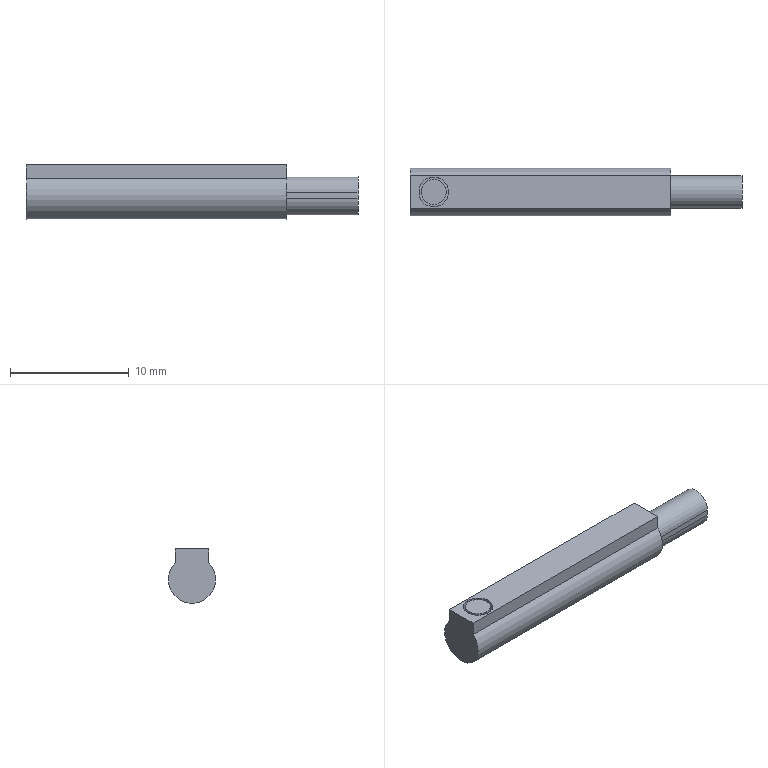Component | SolidWorks | MGPM20-20Z-M9P-1_D_M9P_MGP_Z_6-2 | 1 solid | 17 faces | box 28 x 4 x 4.6 mm | volume 365 mm3 | plane 10 | cylinder 7 | commonest cylinder face diameters 2.7 x2 2.5 x2 2.1 x2 4 x1
STEP:
#1=COLOUR_RGB('',0.7922,0.8196,0.9333);
#2=FILL_AREA_STYLE_COLOUR('',#1);
#3=FILL_AREA_STYLE('',(#2));
#4=SURFACE_STYLE_FILL_AREA(#3);
#5=SURFACE_SIDE_STYLE('',(#4));
#6=SURFACE_STYLE_USAGE(.BOTH.,#5);
#7=PRESENTATION_STYLE_ASSIGNMENT((#6));
#8=CARTESIAN_POINT('',(2.517,1.889,2.967));
#9=VERTEX_POINT('',#8);
#10=CARTESIAN_POINT('',(2.517,1.988,2.967));
#11=VERTEX_POINT('',#10);
#12=CARTESIAN_POINT('',(2.517,1.938,2.967));
#13=DIRECTION('',(0.,0.,1.));
#14=DIRECTION('',(0.,-1.,0.));
#15=AXIS2_PLACEMENT_3D('',#12,#13,#14);
#16=CIRCLE('',#15,0.04921);
#17=EDGE_CURVE('',#9,#11,#16,.T.);
#18=ORIENTED_EDGE('',*,*,#17,.F.);
#19=CARTESIAN_POINT('',(2.517,1.938,2.967));
#20=DIRECTION('',(0.,0.,1.));
#21=DIRECTION('',(0.,-1.,0.));
#22=AXIS2_PLACEMENT_3D('',#19,#20,#21);
#23=CIRCLE('',#22,0.04921);
#24=EDGE_CURVE('',#11,#9,#23,.T.);
#25=ORIENTED_EDGE('',*,*,#24,.F.);
#26=EDGE_LOOP('',(#18,#25));
#27=FACE_BOUND('',#26,.T.);
#28=CARTESIAN_POINT('',(2.438,1.883,2.967));
#29=VERTEX_POINT('',#28);
#30=CARTESIAN_POINT('',(2.438,1.994,2.967));
#31=VERTEX_POINT('',#30);
#32=CARTESIAN_POINT('',(2.438,1.883,2.967));
#33=DIRECTION('',(-0.,1.,-0.));
#34=VECTOR('',#33,39.37);
#35=LINE('',#32,#34);
#36=EDGE_CURVE('',#29,#31,#35,.T.);
#37=ORIENTED_EDGE('',*,*,#36,.F.);
#38=CARTESIAN_POINT('',(3.304,1.883,2.967));
#39=VERTEX_POINT('',#38);
#40=CARTESIAN_POINT('',(3.304,1.883,2.967));
#41=DIRECTION('',(-1.,-0.,0.));
#42=VECTOR('',#41,39.37);
#43=LINE('',#40,#42);
#44=EDGE_CURVE('',#39,#29,#43,.T.);
#45=ORIENTED_EDGE('',*,*,#44,.F.);
#46=CARTESIAN_POINT('',(3.304,1.994,2.967));
#47=VERTEX_POINT('',#46);
#48=CARTESIAN_POINT('',(3.304,1.883,2.967));
#49=DIRECTION('',(-0.,1.,-0.));
#50=VECTOR('',#49,39.37);
#51=LINE('',#48,#50);
#52=EDGE_CURVE('',#39,#47,#51,.T.);
#53=ORIENTED_EDGE('',*,*,#52,.T.);
#54=CARTESIAN_POINT('',(3.304,1.994,2.967));
#55=DIRECTION('',(-1.,-0.,0.));
#56=VECTOR('',#55,39.37);
#57=LINE('',#54,#56);
#58=EDGE_CURVE('',#47,#31,#57,.T.);
#59=ORIENTED_EDGE('',*,*,#58,.T.);
#60=EDGE_LOOP('',(#37,#45,#53,#59));
#61=FACE_OUTER_BOUND('',#60,.T.);
#62=CARTESIAN_POINT('',(3.304,1.883,2.967));
#63=DIRECTION('',(0.,0.,1.));
#64=DIRECTION('',(-1.,-0.,0.));
#65=AXIS2_PLACEMENT_3D('',#62,#63,#64);
#66=PLANE('',#65);
#67=ADVANCED_FACE('',(#27,#61),#66,.T.);
#68=CARTESIAN_POINT('',(2.438,1.994,2.921));
#69=VERTEX_POINT('',#68);
#70=CARTESIAN_POINT('',(2.438,1.994,2.967));
#71=DIRECTION('',(-0.,-0.,-1.));
#72=VECTOR('',#71,39.37);
#73=LINE('',#70,#72);
#74=EDGE_CURVE('',#31,#69,#73,.T.);
#75=ORIENTED_EDGE('',*,*,#74,.F.);
#76=ORIENTED_EDGE('',*,*,#58,.F.);
#77=CARTESIAN_POINT('',(3.304,1.994,2.921));
#78=VERTEX_POINT('',#77);
#79=CARTESIAN_POINT('',(3.304,1.994,2.967));
#80=DIRECTION('',(-0.,-0.,-1.));
#81=VECTOR('',#80,39.37);
#82=LINE('',#79,#81);
#83=EDGE_CURVE('',#47,#78,#82,.T.);
#84=ORIENTED_EDGE('',*,*,#83,.T.);
#85=CARTESIAN_POINT('',(3.304,1.994,2.921));
#86=DIRECTION('',(-1.,-0.,0.));
#87=VECTOR('',#86,39.37);
#88=LINE('',#85,#87);
#89=EDGE_CURVE('',#78,#69,#88,.T.);
#90=ORIENTED_EDGE('',*,*,#89,.T.);
#91=EDGE_LOOP('',(#75,#76,#84,#90));
#92=FACE_OUTER_BOUND('',#91,.T.);
#93=CARTESIAN_POINT('',(3.304,1.994,2.967));
#94=DIRECTION('',(-0.,1.,-0.));
#95=DIRECTION('',(-1.,-0.,0.));
#96=AXIS2_PLACEMENT_3D('',#93,#94,#95);
#97=PLANE('',#96);
#98=ADVANCED_FACE('',(#92),#97,.T.);
#99=CARTESIAN_POINT('',(2.438,1.883,2.921));
#100=VERTEX_POINT('',#99);
#101=CARTESIAN_POINT('',(2.438,1.938,2.865));
#102=DIRECTION('',(-1.,-0.,0.));
#103=DIRECTION('',(0.,-1.,0.));
#104=AXIS2_PLACEMENT_3D('',#101,#102,#103);
#105=CIRCLE('',#104,0.07874);
#106=EDGE_CURVE('',#69,#100,#105,.T.);
#107=ORIENTED_EDGE('',*,*,#106,.F.);
#108=ORIENTED_EDGE('',*,*,#89,.F.);
#109=CARTESIAN_POINT('',(3.304,1.883,2.921));
#110=VERTEX_POINT('',#109);
#111=CARTESIAN_POINT('',(3.304,1.938,2.865));
#112=DIRECTION('',(-1.,-0.,0.));
#113=DIRECTION('',(0.,-1.,0.));
#114=AXIS2_PLACEMENT_3D('',#111,#112,#113);
#115=CIRCLE('',#114,0.07874);
#116=EDGE_CURVE('',#78,#110,#115,.T.);
#117=ORIENTED_EDGE('',*,*,#116,.T.);
#118=CARTESIAN_POINT('',(3.304,1.883,2.921));
#119=DIRECTION('',(-1.,-0.,0.));
#120=VECTOR('',#119,39.37);
#121=LINE('',#118,#120);
#122=EDGE_CURVE('',#110,#100,#121,.T.);
#123=ORIENTED_EDGE('',*,*,#122,.T.);
#124=EDGE_LOOP('',(#107,#108,#117,#123));
#125=FACE_OUTER_BOUND('',#124,.T.);
#126=CARTESIAN_POINT('',(3.304,1.938,2.865));
#127=DIRECTION('',(1.,0.,-0.));
#128=DIRECTION('',(0.,0.,1.));
#129=AXIS2_PLACEMENT_3D('',#126,#127,#128);
#130=CYLINDRICAL_SURFACE('',#129,0.07874);
#131=ADVANCED_FACE('',(#125),#130,.T.);
#132=CARTESIAN_POINT('',(2.438,1.883,2.921));
#133=DIRECTION('',(0.,0.,1.));
#134=VECTOR('',#133,39.37);
#135=LINE('',#132,#134);
#136=EDGE_CURVE('',#100,#29,#135,.T.);
#137=ORIENTED_EDGE('',*,*,#136,.F.);
#138=ORIENTED_EDGE('',*,*,#122,.F.);
#139=CARTESIAN_POINT('',(3.304,1.883,2.921));
#140=DIRECTION('',(0.,0.,1.));
#141=VECTOR('',#140,39.37);
#142=LINE('',#139,#141);
#143=EDGE_CURVE('',#110,#39,#142,.T.);
#144=ORIENTED_EDGE('',*,*,#143,.T.);
#145=ORIENTED_EDGE('',*,*,#44,.T.);
#146=EDGE_LOOP('',(#137,#138,#144,#145));
#147=FACE_OUTER_BOUND('',#146,.T.);
#148=CARTESIAN_POINT('',(3.304,1.883,2.921));
#149=DIRECTION('',(0.,-1.,0.));
#150=DIRECTION('',(1.,0.,-0.));
#151=AXIS2_PLACEMENT_3D('',#148,#149,#150);
#152=PLANE('',#151);
#153=ADVANCED_FACE('',(#147),#152,.T.);
#154=CARTESIAN_POINT('',(3.304,1.885,2.875));
#155=VERTEX_POINT('',#154);
#156=CARTESIAN_POINT('',(3.304,1.992,2.875));
#157=VERTEX_POINT('',#156);
#158=CARTESIAN_POINT('',(3.304,1.938,2.875));
#159=DIRECTION('',(-1.,-0.,0.));
#160=DIRECTION('',(0.,-1.,0.));
#161=AXIS2_PLACEMENT_3D('',#158,#159,#160);
#162=CIRCLE('',#161,0.05315);
#163=EDGE_CURVE('',#155,#157,#162,.T.);
#164=ORIENTED_EDGE('',*,*,#163,.T.);
#165=CARTESIAN_POINT('',(3.304,1.992,2.855));
#166=VERTEX_POINT('',#165);
#167=CARTESIAN_POINT('',(3.304,1.992,2.875));
#168=DIRECTION('',(-0.,-0.,-1.));
#169=VECTOR('',#168,39.37);
#170=LINE('',#167,#169);
#171=EDGE_CURVE('',#157,#166,#170,.T.);
#172=ORIENTED_EDGE('',*,*,#171,.T.);
#173=CARTESIAN_POINT('',(3.304,1.885,2.855));
#174=VERTEX_POINT('',#173);
#175=CARTESIAN_POINT('',(3.304,1.938,2.855));
#176=DIRECTION('',(-1.,-0.,0.));
#177=DIRECTION('',(0.,-1.,0.));
#178=AXIS2_PLACEMENT_3D('',#175,#176,#177);
#179=CIRCLE('',#178,0.05315);
#180=EDGE_CURVE('',#166,#174,#179,.T.);
#181=ORIENTED_EDGE('',*,*,#180,.T.);
#182=CARTESIAN_POINT('',(3.304,1.885,2.855));
#183=DIRECTION('',(0.,0.,1.));
#184=VECTOR('',#183,39.37);
#185=LINE('',#182,#184);
#186=EDGE_CURVE('',#174,#155,#185,.T.);
#187=ORIENTED_EDGE('',*,*,#186,.T.);
#188=EDGE_LOOP('',(#164,#172,#181,#187));
#189=FACE_BOUND('',#188,.T.);
#190=ORIENTED_EDGE('',*,*,#83,.F.);
#191=ORIENTED_EDGE('',*,*,#52,.F.);
#192=ORIENTED_EDGE('',*,*,#143,.F.);
#193=ORIENTED_EDGE('',*,*,#116,.F.);
#194=EDGE_LOOP('',(#190,#191,#192,#193));
#195=FACE_OUTER_BOUND('',#194,.T.);
#196=CARTESIAN_POINT('',(3.304,1.938,2.865));
#197=DIRECTION('',(-1.,-0.,0.));
#198=DIRECTION('',(0.,-1.,0.));
#199=AXIS2_PLACEMENT_3D('',#196,#197,#198);
#200=PLANE('',#199);
#201=ADVANCED_FACE('',(#189,#195),#200,.F.);
#202=ORIENTED_EDGE('',*,*,#186,.F.);
#203=CARTESIAN_POINT('',(3.54,1.885,2.855));
#204=VERTEX_POINT('',#203);
#205=CARTESIAN_POINT('',(3.54,1.885,2.855));
#206=DIRECTION('',(-1.,-0.,0.));
#207=VECTOR('',#206,39.37);
#208=LINE('',#205,#207);
#209=EDGE_CURVE('',#204,#174,#208,.T.);
#210=ORIENTED_EDGE('',*,*,#209,.F.);
#211=CARTESIAN_POINT('',(3.54,1.885,2.875));
#212=VERTEX_POINT('',#211);
#213=CARTESIAN_POINT('',(3.54,1.885,2.855));
#214=DIRECTION('',(0.,0.,1.));
#215=VECTOR('',#214,39.37);
#216=LINE('',#213,#215);
#217=EDGE_CURVE('',#204,#212,#216,.T.);
#218=ORIENTED_EDGE('',*,*,#217,.T.);
#219=CARTESIAN_POINT('',(3.54,1.885,2.875));
#220=DIRECTION('',(-1.,-0.,0.));
#221=VECTOR('',#220,39.37);
#222=LINE('',#219,#221);
#223=EDGE_CURVE('',#212,#155,#222,.T.);
#224=ORIENTED_EDGE('',*,*,#223,.T.);
#225=EDGE_LOOP('',(#202,#210,#218,#224));
#226=FACE_OUTER_BOUND('',#225,.T.);
#227=CARTESIAN_POINT('',(3.54,1.885,2.855));
#228=DIRECTION('',(0.,-1.,0.));
#229=DIRECTION('',(1.,0.,-0.));
#230=AXIS2_PLACEMENT_3D('',#227,#228,#229);
#231=PLANE('',#230);
#232=ADVANCED_FACE('',(#226),#231,.T.);
#233=ORIENTED_EDGE('',*,*,#163,.F.);
#234=ORIENTED_EDGE('',*,*,#223,.F.);
#235=CARTESIAN_POINT('',(3.54,1.992,2.875));
#236=VERTEX_POINT('',#235);
#237=CARTESIAN_POINT('',(3.54,1.938,2.875));
#238=DIRECTION('',(-1.,-0.,0.));
#239=DIRECTION('',(0.,-1.,0.));
#240=AXIS2_PLACEMENT_3D('',#237,#238,#239);
#241=CIRCLE('',#240,0.05315);
#242=EDGE_CURVE('',#212,#236,#241,.T.);
#243=ORIENTED_EDGE('',*,*,#242,.T.);
#244=CARTESIAN_POINT('',(3.54,1.992,2.875));
#245=DIRECTION('',(-1.,-0.,0.));
#246=VECTOR('',#245,39.37);
#247=LINE('',#244,#246);
#248=EDGE_CURVE('',#236,#157,#247,.T.);
#249=ORIENTED_EDGE('',*,*,#248,.T.);
#250=EDGE_LOOP('',(#233,#234,#243,#249));
#251=FACE_OUTER_BOUND('',#250,.T.);
#252=CARTESIAN_POINT('',(3.54,1.938,2.875));
#253=DIRECTION('',(1.,0.,-0.));
#254=DIRECTION('',(0.,0.,-1.));
#255=AXIS2_PLACEMENT_3D('',#252,#253,#254);
#256=CYLINDRICAL_SURFACE('',#255,0.05315);
#257=ADVANCED_FACE('',(#251),#256,.T.);
#258=ORIENTED_EDGE('',*,*,#171,.F.);
#259=ORIENTED_EDGE('',*,*,#248,.F.);
#260=CARTESIAN_POINT('',(3.54,1.992,2.855));
#261=VERTEX_POINT('',#260);
#262=CARTESIAN_POINT('',(3.54,1.992,2.875));
#263=DIRECTION('',(-0.,-0.,-1.));
#264=VECTOR('',#263,39.37);
#265=LINE('',#262,#264);
#266=EDGE_CURVE('',#236,#261,#265,.T.);
#267=ORIENTED_EDGE('',*,*,#266,.T.);
#268=CARTESIAN_POINT('',(3.54,1.992,2.855));
#269=DIRECTION('',(-1.,-0.,0.));
#270=VECTOR('',#269,39.37);
#271=LINE('',#268,#270);
#272=EDGE_CURVE('',#261,#166,#271,.T.);
#273=ORIENTED_EDGE('',*,*,#272,.T.);
#274=EDGE_LOOP('',(#258,#259,#267,#273));
#275=FACE_OUTER_BOUND('',#274,.T.);
#276=CARTESIAN_POINT('',(3.54,1.992,2.875));
#277=DIRECTION('',(-0.,1.,-0.));
#278=DIRECTION('',(-1.,-0.,0.));
#279=AXIS2_PLACEMENT_3D('',#276,#277,#278);
#280=PLANE('',#279);
#281=ADVANCED_FACE('',(#275),#280,.T.);
#282=ORIENTED_EDGE('',*,*,#180,.F.);
#283=ORIENTED_EDGE('',*,*,#272,.F.);
#284=CARTESIAN_POINT('',(3.54,1.938,2.855));
#285=DIRECTION('',(-1.,-0.,0.));
#286=DIRECTION('',(0.,-1.,0.));
#287=AXIS2_PLACEMENT_3D('',#284,#285,#286);
#288=CIRCLE('',#287,0.05315);
#289=EDGE_CURVE('',#261,#204,#288,.T.);
#290=ORIENTED_EDGE('',*,*,#289,.T.);
#291=ORIENTED_EDGE('',*,*,#209,.T.);
#292=EDGE_LOOP('',(#282,#283,#290,#291));
#293=FACE_OUTER_BOUND('',#292,.T.);
#294=CARTESIAN_POINT('',(3.54,1.938,2.855));
#295=DIRECTION('',(1.,0.,-0.));
#296=DIRECTION('',(0.,0.,1.));
#297=AXIS2_PLACEMENT_3D('',#294,#295,#296);
#298=CYLINDRICAL_SURFACE('',#297,0.05315);
#299=ADVANCED_FACE('',(#293),#298,.T.);
#300=ORIENTED_EDGE('',*,*,#266,.F.);
#301=ORIENTED_EDGE('',*,*,#242,.F.);
#302=ORIENTED_EDGE('',*,*,#217,.F.);
#303=ORIENTED_EDGE('',*,*,#289,.F.);
#304=EDGE_LOOP('',(#300,#301,#302,#303));
#305=FACE_OUTER_BOUND('',#304,.T.);
#306=CARTESIAN_POINT('',(3.54,1.938,2.855));
#307=DIRECTION('',(-1.,-0.,0.));
#308=DIRECTION('',(0.,-1.,0.));
#309=AXIS2_PLACEMENT_3D('',#306,#307,#308);
#310=PLANE('',#309);
#311=ADVANCED_FACE('',(#305),#310,.F.);
#312=ORIENTED_EDGE('',*,*,#74,.T.);
#313=ORIENTED_EDGE('',*,*,#106,.T.);
#314=ORIENTED_EDGE('',*,*,#136,.T.);
#315=ORIENTED_EDGE('',*,*,#36,.T.);
#316=EDGE_LOOP('',(#312,#313,#314,#315));
#317=FACE_OUTER_BOUND('',#316,.T.);
#318=CARTESIAN_POINT('',(2.438,1.938,2.865));
#319=DIRECTION('',(-1.,-0.,0.));
#320=DIRECTION('',(0.,-1.,0.));
#321=AXIS2_PLACEMENT_3D('',#318,#319,#320);
#322=PLANE('',#321);
#323=ADVANCED_FACE('',(#317),#322,.T.);
#324=CARTESIAN_POINT('',(2.517,1.988,2.928));
#325=VERTEX_POINT('',#324);
#326=CARTESIAN_POINT('',(2.517,1.889,2.928));
#327=VERTEX_POINT('',#326);
#328=CARTESIAN_POINT('',(2.517,1.938,2.928));
#329=DIRECTION('',(0.,0.,1.));
#330=DIRECTION('',(0.,-1.,0.));
#331=AXIS2_PLACEMENT_3D('',#328,#329,#330);
#332=CIRCLE('',#331,0.04921);
#333=EDGE_CURVE('',#325,#327,#332,.T.);
#334=ORIENTED_EDGE('',*,*,#333,.F.);
#335=CARTESIAN_POINT('',(2.517,1.988,2.967));
#336=DIRECTION('',(-0.,-0.,-1.));
#337=VECTOR('',#336,39.37);
#338=LINE('',#335,#337);
#339=EDGE_CURVE('',#11,#325,#338,.T.);
#340=ORIENTED_EDGE('',*,*,#339,.F.);
#341=ORIENTED_EDGE('',*,*,#24,.T.);
#342=CARTESIAN_POINT('',(2.517,1.889,2.967));
#343=DIRECTION('',(-0.,-0.,-1.));
#344=VECTOR('',#343,39.37);
#345=LINE('',#342,#344);
#346=EDGE_CURVE('',#9,#327,#345,.T.);
#347=ORIENTED_EDGE('',*,*,#346,.T.);
#348=EDGE_LOOP('',(#334,#340,#341,#347));
#349=FACE_OUTER_BOUND('',#348,.T.);
#350=CARTESIAN_POINT('',(2.517,1.938,2.928));
#351=DIRECTION('',(-0.,-0.,-1.));
#352=DIRECTION('',(1.,0.,0.));
#353=AXIS2_PLACEMENT_3D('',#350,#351,#352);
#354=CYLINDRICAL_SURFACE('',#353,0.04921);
#355=ADVANCED_FACE('',(#349),#354,.F.);
#356=ORIENTED_EDGE('',*,*,#17,.T.);
#357=ORIENTED_EDGE('',*,*,#339,.T.);
#358=CARTESIAN_POINT('',(2.517,1.938,2.928));
#359=DIRECTION('',(0.,0.,1.));
#360=DIRECTION('',(0.,-1.,0.));
#361=AXIS2_PLACEMENT_3D('',#358,#359,#360);
#362=CIRCLE('',#361,0.04921);
#363=EDGE_CURVE('',#327,#325,#362,.T.);
#364=ORIENTED_EDGE('',*,*,#363,.F.);
#365=ORIENTED_EDGE('',*,*,#346,.F.);
#366=EDGE_LOOP('',(#356,#357,#364,#365));
#367=FACE_OUTER_BOUND('',#366,.T.);
#368=CARTESIAN_POINT('',(2.517,1.938,2.928));
#369=DIRECTION('',(-0.,-0.,-1.));
#370=DIRECTION('',(-1.,0.,0.));
#371=AXIS2_PLACEMENT_3D('',#368,#369,#370);
#372=CYLINDRICAL_SURFACE('',#371,0.04921);
#373=ADVANCED_FACE('',(#367),#372,.F.);
#374=CARTESIAN_POINT('',(2.517,1.897,2.928));
#375=VERTEX_POINT('',#374);
#376=CARTESIAN_POINT('',(2.517,1.98,2.928));
#377=VERTEX_POINT('',#376);
#378=CARTESIAN_POINT('',(2.517,1.938,2.928));
#379=DIRECTION('',(0.,0.,1.));
#380=DIRECTION('',(0.,-1.,0.));
#381=AXIS2_PLACEMENT_3D('',#378,#379,#380);
#382=CIRCLE('',#381,0.04134);
#383=EDGE_CURVE('',#375,#377,#382,.T.);
#384=ORIENTED_EDGE('',*,*,#383,.F.);
#385=CARTESIAN_POINT('',(2.517,1.938,2.928));
#386=DIRECTION('',(0.,0.,1.));
#387=DIRECTION('',(0.,-1.,0.));
#388=AXIS2_PLACEMENT_3D('',#385,#386,#387);
#389=CIRCLE('',#388,0.04134);
#390=EDGE_CURVE('',#377,#375,#389,.T.);
#391=ORIENTED_EDGE('',*,*,#390,.F.);
#392=EDGE_LOOP('',(#384,#391));
#393=FACE_BOUND('',#392,.T.);
#394=ORIENTED_EDGE('',*,*,#363,.T.);
#395=ORIENTED_EDGE('',*,*,#333,.T.);
#396=EDGE_LOOP('',(#394,#395));
#397=FACE_OUTER_BOUND('',#396,.T.);
#398=CARTESIAN_POINT('',(2.517,1.938,2.928));
#399=DIRECTION('',(0.,0.,1.));
#400=DIRECTION('',(-1.,-0.,0.));
#401=AXIS2_PLACEMENT_3D('',#398,#399,#400);
#402=PLANE('',#401);
#403=ADVANCED_FACE('',(#393,#397),#402,.T.);
#404=ORIENTED_EDGE('',*,*,#390,.T.);
#405=CARTESIAN_POINT('',(2.517,1.897,2.967));
#406=VERTEX_POINT('',#405);
#407=CARTESIAN_POINT('',(2.517,1.897,2.967));
#408=DIRECTION('',(-0.,-0.,-1.));
#409=VECTOR('',#408,39.37);
#410=LINE('',#407,#409);
#411=EDGE_CURVE('',#406,#375,#410,.T.);
#412=ORIENTED_EDGE('',*,*,#411,.F.);
#413=CARTESIAN_POINT('',(2.517,1.98,2.967));
#414=VERTEX_POINT('',#413);
#415=CARTESIAN_POINT('',(2.517,1.938,2.967));
#416=DIRECTION('',(0.,0.,1.));
#417=DIRECTION('',(0.,-1.,0.));
#418=AXIS2_PLACEMENT_3D('',#415,#416,#417);
#419=CIRCLE('',#418,0.04134);
#420=EDGE_CURVE('',#414,#406,#419,.T.);
#421=ORIENTED_EDGE('',*,*,#420,.F.);
#422=CARTESIAN_POINT('',(2.517,1.98,2.967));
#423=DIRECTION('',(-0.,-0.,-1.));
#424=VECTOR('',#423,39.37);
#425=LINE('',#422,#424);
#426=EDGE_CURVE('',#414,#377,#425,.T.);
#427=ORIENTED_EDGE('',*,*,#426,.T.);
#428=EDGE_LOOP('',(#404,#412,#421,#427));
#429=FACE_OUTER_BOUND('',#428,.T.);
#430=CARTESIAN_POINT('',(2.517,1.938,2.928));
#431=DIRECTION('',(-0.,-0.,-1.));
#432=DIRECTION('',(1.,0.,0.));
#433=AXIS2_PLACEMENT_3D('',#430,#431,#432);
#434=CYLINDRICAL_SURFACE('',#433,0.04134);
#435=ADVANCED_FACE('',(#429),#434,.T.);
#436=CARTESIAN_POINT('',(2.517,1.938,2.967));
#437=DIRECTION('',(0.,0.,1.));
#438=DIRECTION('',(0.,-1.,0.));
#439=AXIS2_PLACEMENT_3D('',#436,#437,#438);
#440=CIRCLE('',#439,0.04134);
#441=EDGE_CURVE('',#406,#414,#440,.T.);
#442=ORIENTED_EDGE('',*,*,#441,.F.);
#443=ORIENTED_EDGE('',*,*,#411,.T.);
#444=ORIENTED_EDGE('',*,*,#383,.T.);
#445=ORIENTED_EDGE('',*,*,#426,.F.);
#446=EDGE_LOOP('',(#442,#443,#444,#445));
#447=FACE_OUTER_BOUND('',#446,.T.);
#448=CARTESIAN_POINT('',(2.517,1.938,2.928));
#449=DIRECTION('',(-0.,-0.,-1.));
#450=DIRECTION('',(-1.,0.,0.));
#451=AXIS2_PLACEMENT_3D('',#448,#449,#450);
#452=CYLINDRICAL_SURFACE('',#451,0.04134);
#453=ADVANCED_FACE('',(#447),#452,.T.);
#454=ORIENTED_EDGE('',*,*,#441,.T.);
#455=ORIENTED_EDGE('',*,*,#420,.T.);
#456=EDGE_LOOP('',(#454,#455));
#457=FACE_OUTER_BOUND('',#456,.T.);
#458=CARTESIAN_POINT('',(3.304,1.883,2.967));
#459=DIRECTION('',(0.,0.,1.));
#460=DIRECTION('',(-1.,-0.,0.));
#461=AXIS2_PLACEMENT_3D('',#458,#459,#460);
#462=PLANE('',#461);
#463=ADVANCED_FACE('',(#457),#462,.T.);
#464=CLOSED_SHELL('',(#67,#98,#131,#153,#201,#232,#257,#281,#299,#311,#323,#355,#373,#403,#435,#453,#463));
#465=MANIFOLD_SOLID_BREP('',#464);
#466=STYLED_ITEM('',(#7),#465);
#467=(LENGTH_UNIT()NAMED_UNIT(*)SI_UNIT($,.METRE.));
#468=LENGTH_MEASURE_WITH_UNIT(LENGTH_MEASURE(0.0254),#467);
#469=DIMENSIONAL_EXPONENTS(1.,0.,0.,0.,0.,0.,0.);
#470=(CONVERSION_BASED_UNIT('',#468)LENGTH_UNIT()NAMED_UNIT(#469));
#471=UNCERTAINTY_MEASURE_WITH_UNIT(LENGTH_MEASURE(0.00001),#470,'','');
#472=(NAMED_UNIT(*)PLANE_ANGLE_UNIT()SI_UNIT($,.RADIAN.));
#473=(NAMED_UNIT(*)SI_UNIT($,.STERADIAN.)SOLID_ANGLE_UNIT());
#474=(GEOMETRIC_REPRESENTATION_CONTEXT(3)GLOBAL_UNCERTAINTY_ASSIGNED_CONTEXT((#471))GLOBAL_UNIT_ASSIGNED_CONTEXT((#470,#472,#473))REPRESENTATION_CONTEXT('',''));
#475=MECHANICAL_DESIGN_GEOMETRIC_PRESENTATION_REPRESENTATION('',(#466),#474);
#476=CARTESIAN_POINT('',(0.,0.,0.));
#477=DIRECTION('',(0.,0.,1.));
#478=DIRECTION('',(1.,0.,0.));
#479=AXIS2_PLACEMENT_3D('',#476,#477,#478);
#480=(LENGTH_UNIT()NAMED_UNIT(*)SI_UNIT($,.METRE.));
#481=LENGTH_MEASURE_WITH_UNIT(LENGTH_MEASURE(0.0254),#480);
#482=DIMENSIONAL_EXPONENTS(1.,0.,0.,0.,0.,0.,0.);
#483=(CONVERSION_BASED_UNIT('',#481)LENGTH_UNIT()NAMED_UNIT(#482));
#484=UNCERTAINTY_MEASURE_WITH_UNIT(LENGTH_MEASURE(0.00001),#483,'','');
#485=(NAMED_UNIT(*)PLANE_ANGLE_UNIT()SI_UNIT($,.RADIAN.));
#486=(NAMED_UNIT(*)SI_UNIT($,.STERADIAN.)SOLID_ANGLE_UNIT());
#487=(GEOMETRIC_REPRESENTATION_CONTEXT(3)GLOBAL_UNCERTAINTY_ASSIGNED_CONTEXT((#484))GLOBAL_UNIT_ASSIGNED_CONTEXT((#483,#485,#486))REPRESENTATION_CONTEXT('',''));
#488=ADVANCED_BREP_SHAPE_REPRESENTATION('',(#465,#479),#487);
#489=PRESENTATION_LAYER_ASSIGNMENT('','',(#466));